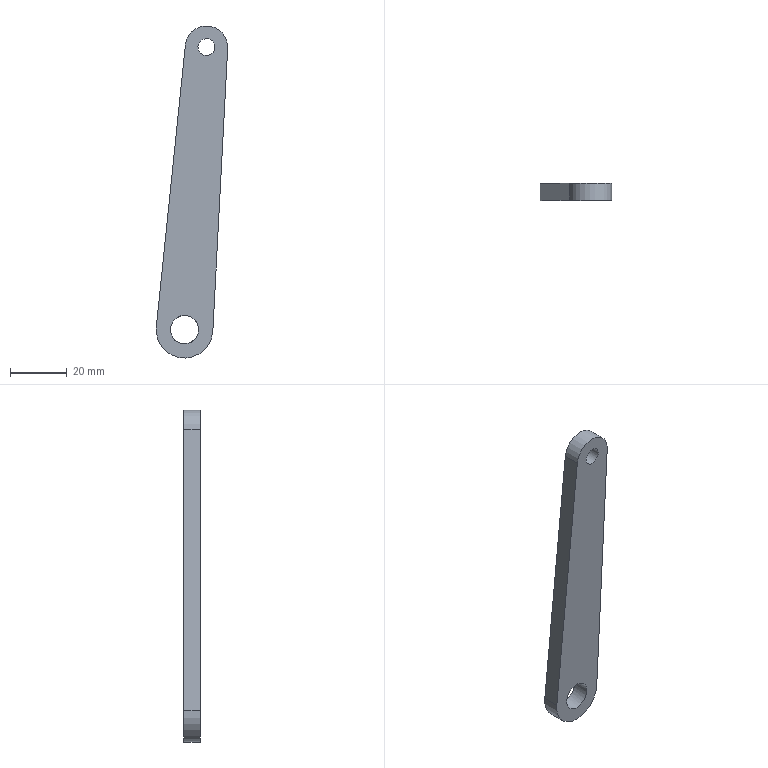Component | NX | CONNECTING_ROD | 1 solid | 8 faces | box 25.25 x 6 x 117.2 mm | volume 11335 mm3 | plane 4 | cylinder 4 | commonest cylinder face diameters 20 x1 15 x1 10 x1 6 x1
STEP:
#1=CARTESIAN_POINT('',(0.,0.,0.));
#2=DIRECTION('',(0.,0.,1.));
#3=DIRECTION('',(1.,0.,0.));
#4=AXIS2_PLACEMENT_3D('',#1,#2,#3);
#5=CARTESIAN_POINT('',(-7.355,48.,110.703));
#6=VERTEX_POINT('',#5);
#7=CARTESIAN_POINT('',(-17.588,48.,11.259));
#8=VERTEX_POINT('',#7);
#9=CARTESIAN_POINT('',(-7.355,48.,110.703));
#10=DIRECTION('',(-0.1024,0.,-0.9947));
#11=VECTOR('',#10,1.);
#12=LINE('',#9,#11);
#13=CARTESIAN_POINT('',(-7.355,42.,110.703));
#14=DIRECTION('',(0.9947,0.,-0.1024));
#15=DIRECTION('',(-0.1024,0.,-0.9947));
#16=AXIS2_PLACEMENT_3D('',#13,#14,#15);
#17=PLANE('',#16);
#18=CARTESIAN_POINT('',(0.,6.));
#19=DIRECTION('',(1.,0.));
#20=VECTOR('',#19,1.);
#21=LINE('',#18,#20);
#22=(GEOMETRIC_REPRESENTATION_CONTEXT(2)PARAMETRIC_REPRESENTATION_CONTEXT()REPRESENTATION_CONTEXT('',''));
#23=DEFINITIONAL_REPRESENTATION('',(#21),#22);
#24=PCURVE('',#17,#23);
#25=CARTESIAN_POINT('',(-7.64,48.,10.235));
#26=DIRECTION('',(0.,-1.,0.));
#27=DIRECTION('',(-0.07746,0.,-0.997));
#28=AXIS2_PLACEMENT_3D('',#25,#26,#27);
#29=PLANE('',#28);
#30=CARTESIAN_POINT('',(-100.188,-7.498));
#31=DIRECTION('',(0.9997,-0.025));
#32=VECTOR('',#31,1.);
#33=LINE('',#30,#32);
#34=(GEOMETRIC_REPRESENTATION_CONTEXT(2)PARAMETRIC_REPRESENTATION_CONTEXT()REPRESENTATION_CONTEXT('',''));
#35=DEFINITIONAL_REPRESENTATION('',(#33),#34);
#36=PCURVE('',#29,#35);
#37=SURFACE_CURVE('',#12,(#24,#36),.PCURVE_S1.);
#38=EDGE_CURVE('',#6,#8,#37,.T.);
#39=ORIENTED_EDGE('',*,*,#38,.T.);
#40=CARTESIAN_POINT('',(-17.588,42.,11.259));
#41=VERTEX_POINT('',#40);
#42=CARTESIAN_POINT('',(-17.588,42.,11.259));
#43=DIRECTION('',(0.,1.,0.));
#44=VECTOR('',#43,1.);
#45=LINE('',#42,#44);
#46=CARTESIAN_POINT('',(99.969,0.));
#47=DIRECTION('',(0.,1.));
#48=VECTOR('',#47,1.);
#49=LINE('',#46,#48);
#50=(GEOMETRIC_REPRESENTATION_CONTEXT(2)PARAMETRIC_REPRESENTATION_CONTEXT()REPRESENTATION_CONTEXT('',''));
#51=DEFINITIONAL_REPRESENTATION('',(#49),#50);
#52=PCURVE('',#17,#51);
#53=CARTESIAN_POINT('',(-7.64,42.,10.235));
#54=DIRECTION('',(0.,1.,0.));
#55=DIRECTION('',(0.07746,0.,0.997));
#56=AXIS2_PLACEMENT_3D('',#53,#54,#55);
#57=CYLINDRICAL_SURFACE('',#56,10.);
#58=CARTESIAN_POINT('',(4.737,0.));
#59=DIRECTION('',(0.,1.));
#60=VECTOR('',#59,1.);
#61=LINE('',#58,#60);
#62=(GEOMETRIC_REPRESENTATION_CONTEXT(2)PARAMETRIC_REPRESENTATION_CONTEXT()REPRESENTATION_CONTEXT('',''));
#63=DEFINITIONAL_REPRESENTATION('',(#61),#62);
#64=PCURVE('',#57,#63);
#65=SURFACE_CURVE('',#45,(#52,#64),.PCURVE_S1.);
#66=EDGE_CURVE('',#41,#8,#65,.T.);
#67=ORIENTED_EDGE('',*,*,#66,.F.);
#68=CARTESIAN_POINT('',(-7.355,42.,110.703));
#69=VERTEX_POINT('',#68);
#70=CARTESIAN_POINT('',(-7.355,42.,110.703));
#71=DIRECTION('',(-0.1024,0.,-0.9947));
#72=VECTOR('',#71,1.);
#73=LINE('',#70,#72);
#74=CARTESIAN_POINT('',(0.,0.));
#75=DIRECTION('',(1.,0.));
#76=VECTOR('',#75,1.);
#77=LINE('',#74,#76);
#78=(GEOMETRIC_REPRESENTATION_CONTEXT(2)PARAMETRIC_REPRESENTATION_CONTEXT()REPRESENTATION_CONTEXT('',''));
#79=DEFINITIONAL_REPRESENTATION('',(#77),#78);
#80=PCURVE('',#17,#79);
#81=CARTESIAN_POINT('',(-7.64,42.,10.235));
#82=DIRECTION('',(0.,-1.,0.));
#83=DIRECTION('',(-0.07746,0.,-0.997));
#84=AXIS2_PLACEMENT_3D('',#81,#82,#83);
#85=PLANE('',#84);
#86=CARTESIAN_POINT('',(-100.188,-7.498));
#87=DIRECTION('',(0.9997,-0.025));
#88=VECTOR('',#87,1.);
#89=LINE('',#86,#88);
#90=(GEOMETRIC_REPRESENTATION_CONTEXT(2)PARAMETRIC_REPRESENTATION_CONTEXT()REPRESENTATION_CONTEXT('',''));
#91=DEFINITIONAL_REPRESENTATION('',(#89),#90);
#92=PCURVE('',#85,#91);
#93=SURFACE_CURVE('',#73,(#80,#92),.PCURVE_S1.);
#94=EDGE_CURVE('',#69,#41,#93,.T.);
#95=ORIENTED_EDGE('',*,*,#94,.F.);
#96=CARTESIAN_POINT('',(-7.355,42.,110.703));
#97=DIRECTION('',(0.,1.,0.));
#98=VECTOR('',#97,1.);
#99=LINE('',#96,#98);
#100=CARTESIAN_POINT('',(0.,0.));
#101=DIRECTION('',(0.,1.));
#102=VECTOR('',#101,1.);
#103=LINE('',#100,#102);
#104=(GEOMETRIC_REPRESENTATION_CONTEXT(2)PARAMETRIC_REPRESENTATION_CONTEXT()REPRESENTATION_CONTEXT('',''));
#105=DEFINITIONAL_REPRESENTATION('',(#103),#104);
#106=PCURVE('',#17,#105);
#107=CARTESIAN_POINT('',(0.1056,42.,109.935));
#108=DIRECTION('',(0.,1.,0.));
#109=DIRECTION('',(0.07746,0.,0.997));
#110=AXIS2_PLACEMENT_3D('',#107,#108,#109);
#111=CYLINDRICAL_SURFACE('',#110,7.5);
#112=CARTESIAN_POINT('',(-1.546,0.));
#113=DIRECTION('',(0.,1.));
#114=VECTOR('',#113,1.);
#115=LINE('',#112,#114);
#116=(GEOMETRIC_REPRESENTATION_CONTEXT(2)PARAMETRIC_REPRESENTATION_CONTEXT()REPRESENTATION_CONTEXT('',''));
#117=DEFINITIONAL_REPRESENTATION('',(#115),#116);
#118=PCURVE('',#111,#117);
#119=SURFACE_CURVE('',#99,(#106,#118),.PCURVE_S1.);
#120=EDGE_CURVE('',#69,#6,#119,.T.);
#121=ORIENTED_EDGE('',*,*,#120,.T.);
#122=EDGE_LOOP('',(#39,#67,#95,#121));
#123=FACE_BOUND('',#122,.T.);
#124=ADVANCED_FACE('',(#123),#17,.F.);
#125=CARTESIAN_POINT('',(2.346,48.,9.71));
#126=VERTEX_POINT('',#125);
#127=CARTESIAN_POINT('',(-7.64,48.,10.235));
#128=DIRECTION('',(0.,-1.,0.));
#129=DIRECTION('',(0.997,0.,-0.07746));
#130=AXIS2_PLACEMENT_3D('',#127,#128,#129);
#131=CIRCLE('',#130,10.);
#132=CARTESIAN_POINT('',(7.854,6.));
#133=DIRECTION('',(-1.,0.));
#134=VECTOR('',#133,1.);
#135=LINE('',#132,#134);
#136=(GEOMETRIC_REPRESENTATION_CONTEXT(2)PARAMETRIC_REPRESENTATION_CONTEXT()REPRESENTATION_CONTEXT('',''));
#137=DEFINITIONAL_REPRESENTATION('',(#135),#136);
#138=PCURVE('',#57,#137);
#139=CARTESIAN_POINT('',(0.,0.));
#140=DIRECTION('',(0.,1.));
#141=AXIS2_PLACEMENT_2D('',#139,#140);
#142=CIRCLE('',#141,10.);
#143=(GEOMETRIC_REPRESENTATION_CONTEXT(2)PARAMETRIC_REPRESENTATION_CONTEXT()REPRESENTATION_CONTEXT('',''));
#144=DEFINITIONAL_REPRESENTATION('',(#142),#143);
#145=PCURVE('',#29,#144);
#146=SURFACE_CURVE('',#131,(#138,#145),.PCURVE_S1.);
#147=EDGE_CURVE('',#8,#126,#146,.T.);
#148=ORIENTED_EDGE('',*,*,#147,.T.);
#149=CARTESIAN_POINT('',(2.346,42.,9.71));
#150=VERTEX_POINT('',#149);
#151=CARTESIAN_POINT('',(2.346,42.,9.71));
#152=DIRECTION('',(0.,1.,0.));
#153=VECTOR('',#152,1.);
#154=LINE('',#151,#153);
#155=CARTESIAN_POINT('',(1.546,0.));
#156=DIRECTION('',(0.,1.));
#157=VECTOR('',#156,1.);
#158=LINE('',#155,#157);
#159=(GEOMETRIC_REPRESENTATION_CONTEXT(2)PARAMETRIC_REPRESENTATION_CONTEXT()REPRESENTATION_CONTEXT('',''));
#160=DEFINITIONAL_REPRESENTATION('',(#158),#159);
#161=PCURVE('',#57,#160);
#162=CARTESIAN_POINT('',(2.346,42.,9.71));
#163=DIRECTION('',(-0.9986,0.,0.05251));
#164=DIRECTION('',(0.05251,0.,0.9986));
#165=AXIS2_PLACEMENT_3D('',#162,#163,#164);
#166=PLANE('',#165);
#167=CARTESIAN_POINT('',(0.,0.));
#168=DIRECTION('',(0.,1.));
#169=VECTOR('',#168,1.);
#170=LINE('',#167,#169);
#171=(GEOMETRIC_REPRESENTATION_CONTEXT(2)PARAMETRIC_REPRESENTATION_CONTEXT()REPRESENTATION_CONTEXT('',''));
#172=DEFINITIONAL_REPRESENTATION('',(#170),#171);
#173=PCURVE('',#166,#172);
#174=SURFACE_CURVE('',#154,(#161,#173),.PCURVE_S1.);
#175=EDGE_CURVE('',#150,#126,#174,.T.);
#176=ORIENTED_EDGE('',*,*,#175,.F.);
#177=CARTESIAN_POINT('',(-7.64,42.,10.235));
#178=DIRECTION('',(0.,-1.,0.));
#179=DIRECTION('',(0.997,0.,-0.07746));
#180=AXIS2_PLACEMENT_3D('',#177,#178,#179);
#181=CIRCLE('',#180,10.);
#182=CARTESIAN_POINT('',(7.854,0.));
#183=DIRECTION('',(-1.,0.));
#184=VECTOR('',#183,1.);
#185=LINE('',#182,#184);
#186=(GEOMETRIC_REPRESENTATION_CONTEXT(2)PARAMETRIC_REPRESENTATION_CONTEXT()REPRESENTATION_CONTEXT('',''));
#187=DEFINITIONAL_REPRESENTATION('',(#185),#186);
#188=PCURVE('',#57,#187);
#189=CARTESIAN_POINT('',(0.,0.));
#190=DIRECTION('',(0.,1.));
#191=AXIS2_PLACEMENT_2D('',#189,#190);
#192=CIRCLE('',#191,10.);
#193=(GEOMETRIC_REPRESENTATION_CONTEXT(2)PARAMETRIC_REPRESENTATION_CONTEXT()REPRESENTATION_CONTEXT('',''));
#194=DEFINITIONAL_REPRESENTATION('',(#192),#193);
#195=PCURVE('',#85,#194);
#196=SURFACE_CURVE('',#181,(#188,#195),.PCURVE_S1.);
#197=EDGE_CURVE('',#41,#150,#196,.T.);
#198=ORIENTED_EDGE('',*,*,#197,.F.);
#199=ORIENTED_EDGE('',*,*,#66,.T.);
#200=EDGE_LOOP('',(#148,#176,#198,#199));
#201=FACE_BOUND('',#200,.T.);
#202=ADVANCED_FACE('',(#201),#57,.T.);
#203=CARTESIAN_POINT('',(7.595,48.,109.541));
#204=VERTEX_POINT('',#203);
#205=CARTESIAN_POINT('',(2.346,48.,9.71));
#206=DIRECTION('',(0.05251,0.,0.9986));
#207=VECTOR('',#206,1.);
#208=LINE('',#205,#207);
#209=CARTESIAN_POINT('',(0.,6.));
#210=DIRECTION('',(1.,0.));
#211=VECTOR('',#210,1.);
#212=LINE('',#209,#211);
#213=(GEOMETRIC_REPRESENTATION_CONTEXT(2)PARAMETRIC_REPRESENTATION_CONTEXT()REPRESENTATION_CONTEXT('',''));
#214=DEFINITIONAL_REPRESENTATION('',(#212),#213);
#215=PCURVE('',#166,#214);
#216=CARTESIAN_POINT('',(-0.25,9.997));
#217=DIRECTION('',(-0.9997,-0.025));
#218=VECTOR('',#217,1.);
#219=LINE('',#216,#218);
#220=(GEOMETRIC_REPRESENTATION_CONTEXT(2)PARAMETRIC_REPRESENTATION_CONTEXT()REPRESENTATION_CONTEXT('',''));
#221=DEFINITIONAL_REPRESENTATION('',(#219),#220);
#222=PCURVE('',#29,#221);
#223=SURFACE_CURVE('',#208,(#215,#222),.PCURVE_S1.);
#224=EDGE_CURVE('',#126,#204,#223,.T.);
#225=ORIENTED_EDGE('',*,*,#224,.T.);
#226=CARTESIAN_POINT('',(7.595,42.,109.541));
#227=VERTEX_POINT('',#226);
#228=CARTESIAN_POINT('',(7.595,42.,109.541));
#229=DIRECTION('',(0.,1.,0.));
#230=VECTOR('',#229,1.);
#231=LINE('',#228,#230);
#232=CARTESIAN_POINT('',(99.969,0.));
#233=DIRECTION('',(0.,1.));
#234=VECTOR('',#233,1.);
#235=LINE('',#232,#234);
#236=(GEOMETRIC_REPRESENTATION_CONTEXT(2)PARAMETRIC_REPRESENTATION_CONTEXT()REPRESENTATION_CONTEXT('',''));
#237=DEFINITIONAL_REPRESENTATION('',(#235),#236);
#238=PCURVE('',#166,#237);
#239=CARTESIAN_POINT('',(1.546,0.));
#240=DIRECTION('',(0.,1.));
#241=VECTOR('',#240,1.);
#242=LINE('',#239,#241);
#243=(GEOMETRIC_REPRESENTATION_CONTEXT(2)PARAMETRIC_REPRESENTATION_CONTEXT()REPRESENTATION_CONTEXT('',''));
#244=DEFINITIONAL_REPRESENTATION('',(#242),#243);
#245=PCURVE('',#111,#244);
#246=SURFACE_CURVE('',#231,(#238,#245),.PCURVE_S1.);
#247=EDGE_CURVE('',#227,#204,#246,.T.);
#248=ORIENTED_EDGE('',*,*,#247,.F.);
#249=CARTESIAN_POINT('',(2.346,42.,9.71));
#250=DIRECTION('',(0.05251,0.,0.9986));
#251=VECTOR('',#250,1.);
#252=LINE('',#249,#251);
#253=CARTESIAN_POINT('',(0.,0.));
#254=DIRECTION('',(1.,0.));
#255=VECTOR('',#254,1.);
#256=LINE('',#253,#255);
#257=(GEOMETRIC_REPRESENTATION_CONTEXT(2)PARAMETRIC_REPRESENTATION_CONTEXT()REPRESENTATION_CONTEXT('',''));
#258=DEFINITIONAL_REPRESENTATION('',(#256),#257);
#259=PCURVE('',#166,#258);
#260=CARTESIAN_POINT('',(-0.25,9.997));
#261=DIRECTION('',(-0.9997,-0.025));
#262=VECTOR('',#261,1.);
#263=LINE('',#260,#262);
#264=(GEOMETRIC_REPRESENTATION_CONTEXT(2)PARAMETRIC_REPRESENTATION_CONTEXT()REPRESENTATION_CONTEXT('',''));
#265=DEFINITIONAL_REPRESENTATION('',(#263),#264);
#266=PCURVE('',#85,#265);
#267=SURFACE_CURVE('',#252,(#259,#266),.PCURVE_S1.);
#268=EDGE_CURVE('',#150,#227,#267,.T.);
#269=ORIENTED_EDGE('',*,*,#268,.F.);
#270=ORIENTED_EDGE('',*,*,#175,.T.);
#271=EDGE_LOOP('',(#225,#248,#269,#270));
#272=FACE_BOUND('',#271,.T.);
#273=ADVANCED_FACE('',(#272),#166,.F.);
#274=CARTESIAN_POINT('',(0.1056,48.,109.935));
#275=DIRECTION('',(0.,-1.,0.));
#276=DIRECTION('',(0.997,0.,-0.07746));
#277=AXIS2_PLACEMENT_3D('',#274,#275,#276);
#278=CIRCLE('',#277,7.5);
#279=CARTESIAN_POINT('',(1.571,6.));
#280=DIRECTION('',(-1.,0.));
#281=VECTOR('',#280,1.);
#282=LINE('',#279,#281);
#283=(GEOMETRIC_REPRESENTATION_CONTEXT(2)PARAMETRIC_REPRESENTATION_CONTEXT()REPRESENTATION_CONTEXT('',''));
#284=DEFINITIONAL_REPRESENTATION('',(#282),#283);
#285=PCURVE('',#111,#284);
#286=CARTESIAN_POINT('',(-100.,0.));
#287=DIRECTION('',(-0.,1.));
#288=AXIS2_PLACEMENT_2D('',#286,#287);
#289=CIRCLE('',#288,7.5);
#290=(GEOMETRIC_REPRESENTATION_CONTEXT(2)PARAMETRIC_REPRESENTATION_CONTEXT()REPRESENTATION_CONTEXT('',''));
#291=DEFINITIONAL_REPRESENTATION('',(#289),#290);
#292=PCURVE('',#29,#291);
#293=SURFACE_CURVE('',#278,(#285,#292),.PCURVE_S1.);
#294=EDGE_CURVE('',#204,#6,#293,.T.);
#295=ORIENTED_EDGE('',*,*,#294,.T.);
#296=ORIENTED_EDGE('',*,*,#120,.F.);
#297=CARTESIAN_POINT('',(0.1056,42.,109.935));
#298=DIRECTION('',(0.,-1.,0.));
#299=DIRECTION('',(0.997,0.,-0.07746));
#300=AXIS2_PLACEMENT_3D('',#297,#298,#299);
#301=CIRCLE('',#300,7.5);
#302=CARTESIAN_POINT('',(1.571,0.));
#303=DIRECTION('',(-1.,0.));
#304=VECTOR('',#303,1.);
#305=LINE('',#302,#304);
#306=(GEOMETRIC_REPRESENTATION_CONTEXT(2)PARAMETRIC_REPRESENTATION_CONTEXT()REPRESENTATION_CONTEXT('',''));
#307=DEFINITIONAL_REPRESENTATION('',(#305),#306);
#308=PCURVE('',#111,#307);
#309=CARTESIAN_POINT('',(-100.,0.));
#310=DIRECTION('',(-0.,1.));
#311=AXIS2_PLACEMENT_2D('',#309,#310);
#312=CIRCLE('',#311,7.5);
#313=(GEOMETRIC_REPRESENTATION_CONTEXT(2)PARAMETRIC_REPRESENTATION_CONTEXT()REPRESENTATION_CONTEXT('',''));
#314=DEFINITIONAL_REPRESENTATION('',(#312),#313);
#315=PCURVE('',#85,#314);
#316=SURFACE_CURVE('',#301,(#308,#315),.PCURVE_S1.);
#317=EDGE_CURVE('',#227,#69,#316,.T.);
#318=ORIENTED_EDGE('',*,*,#317,.F.);
#319=ORIENTED_EDGE('',*,*,#247,.T.);
#320=EDGE_LOOP('',(#295,#296,#318,#319));
#321=FACE_BOUND('',#320,.T.);
#322=ADVANCED_FACE('',(#321),#111,.T.);
#323=CARTESIAN_POINT('',(-0.1268,42.,106.944));
#324=VERTEX_POINT('',#323);
#325=CARTESIAN_POINT('',(-2.885,42.,110.167));
#326=VERTEX_POINT('',#325);
#327=CARTESIAN_POINT('',(0.1056,42.,109.935));
#328=DIRECTION('',(0.,1.,0.));
#329=DIRECTION('',(-0.07746,0.,-0.997));
#330=AXIS2_PLACEMENT_3D('',#327,#328,#329);
#331=CIRCLE('',#330,3.);
#332=CARTESIAN_POINT('',(-97.,0.));
#333=CARTESIAN_POINT('',(-97.,-5.196));
#334=CARTESIAN_POINT('',(-101.5,-2.598));
#335=CARTESIAN_POINT('',(-106.,0.));
#336=CARTESIAN_POINT('',(-101.5,2.598));
#337=CARTESIAN_POINT('',(-97.,5.196));
#338=CARTESIAN_POINT('',(-97.,0.));
#339=(BOUNDED_CURVE()B_SPLINE_CURVE(2,(#332,#333,#334,#335,#336,#337,#338),.UNSPECIFIED.,.T.,.F.)B_SPLINE_CURVE_WITH_KNOTS((1,2,2,2,2,1),(-2.094,0.,2.094,4.189,6.283,8.378),.UNSPECIFIED.)CURVE()GEOMETRIC_REPRESENTATION_ITEM()RATIONAL_B_SPLINE_CURVE((1.,0.5,1.,0.5,1.,0.5,1.))REPRESENTATION_ITEM(''));
#340=(GEOMETRIC_REPRESENTATION_CONTEXT(2)PARAMETRIC_REPRESENTATION_CONTEXT()REPRESENTATION_CONTEXT('',''));
#341=DEFINITIONAL_REPRESENTATION('',(#339),#340);
#342=PCURVE('',#85,#341);
#343=CARTESIAN_POINT('',(0.1056,41.4,109.935));
#344=DIRECTION('',(0.,1.,0.));
#345=DIRECTION('',(0.07746,0.,0.997));
#346=AXIS2_PLACEMENT_3D('',#343,#344,#345);
#347=CYLINDRICAL_SURFACE('',#346,3.);
#348=CARTESIAN_POINT('',(9.425,0.6));
#349=DIRECTION('',(1.,0.));
#350=VECTOR('',#349,1.);
#351=LINE('',#348,#350);
#352=(GEOMETRIC_REPRESENTATION_CONTEXT(2)PARAMETRIC_REPRESENTATION_CONTEXT()REPRESENTATION_CONTEXT('',''));
#353=DEFINITIONAL_REPRESENTATION('',(#351),#352);
#354=PCURVE('',#347,#353);
#355=SURFACE_CURVE('',#331,(#342,#354),.PCURVE_S1.);
#356=EDGE_CURVE('',#324,#326,#355,.T.);
#357=ORIENTED_EDGE('',*,*,#356,.T.);
#358=CARTESIAN_POINT('',(0.1056,42.,109.935));
#359=DIRECTION('',(0.,1.,0.));
#360=DIRECTION('',(-0.07746,0.,-0.997));
#361=AXIS2_PLACEMENT_3D('',#358,#359,#360);
#362=CIRCLE('',#361,3.);
#363=CARTESIAN_POINT('',(-97.,0.));
#364=CARTESIAN_POINT('',(-97.,-5.196));
#365=CARTESIAN_POINT('',(-101.5,-2.598));
#366=CARTESIAN_POINT('',(-106.,0.));
#367=CARTESIAN_POINT('',(-101.5,2.598));
#368=CARTESIAN_POINT('',(-97.,5.196));
#369=CARTESIAN_POINT('',(-97.,0.));
#370=(BOUNDED_CURVE()B_SPLINE_CURVE(2,(#363,#364,#365,#366,#367,#368,#369),.UNSPECIFIED.,.T.,.F.)B_SPLINE_CURVE_WITH_KNOTS((1,2,2,2,2,1),(-2.094,0.,2.094,4.189,6.283,8.378),.UNSPECIFIED.)CURVE()GEOMETRIC_REPRESENTATION_ITEM()RATIONAL_B_SPLINE_CURVE((1.,0.5,1.,0.5,1.,0.5,1.))REPRESENTATION_ITEM(''));
#371=(GEOMETRIC_REPRESENTATION_CONTEXT(2)PARAMETRIC_REPRESENTATION_CONTEXT()REPRESENTATION_CONTEXT('',''));
#372=DEFINITIONAL_REPRESENTATION('',(#370),#371);
#373=PCURVE('',#85,#372);
#374=CARTESIAN_POINT('',(3.142,0.6));
#375=DIRECTION('',(1.,0.));
#376=VECTOR('',#375,1.);
#377=LINE('',#374,#376);
#378=(GEOMETRIC_REPRESENTATION_CONTEXT(2)PARAMETRIC_REPRESENTATION_CONTEXT()REPRESENTATION_CONTEXT('',''));
#379=DEFINITIONAL_REPRESENTATION('',(#377),#378);
#380=PCURVE('',#347,#379);
#381=SURFACE_CURVE('',#362,(#373,#380),.PCURVE_S1.);
#382=EDGE_CURVE('',#326,#324,#381,.T.);
#383=ORIENTED_EDGE('',*,*,#382,.T.);
#384=EDGE_LOOP('',(#357,#383));
#385=FACE_BOUND('',#384,.T.);
#386=CARTESIAN_POINT('',(-8.027,42.,5.25));
#387=VERTEX_POINT('',#386);
#388=CARTESIAN_POINT('',(-12.625,42.,10.623));
#389=VERTEX_POINT('',#388);
#390=CARTESIAN_POINT('',(-7.64,42.,10.235));
#391=DIRECTION('',(0.,1.,0.));
#392=DIRECTION('',(-0.07746,0.,-0.997));
#393=AXIS2_PLACEMENT_3D('',#390,#391,#392);
#394=CIRCLE('',#393,5.);
#395=CARTESIAN_POINT('',(5.,0.));
#396=CARTESIAN_POINT('',(5.,-8.66));
#397=CARTESIAN_POINT('',(-2.5,-4.33));
#398=CARTESIAN_POINT('',(-10.,-0.));
#399=CARTESIAN_POINT('',(-2.5,4.33));
#400=CARTESIAN_POINT('',(5.,8.66));
#401=CARTESIAN_POINT('',(5.,0.));
#402=(BOUNDED_CURVE()B_SPLINE_CURVE(2,(#395,#396,#397,#398,#399,#400,#401),.UNSPECIFIED.,.T.,.F.)B_SPLINE_CURVE_WITH_KNOTS((1,2,2,2,2,1),(-2.094,0.,2.094,4.189,6.283,8.378),.UNSPECIFIED.)CURVE()GEOMETRIC_REPRESENTATION_ITEM()RATIONAL_B_SPLINE_CURVE((1.,0.5,1.,0.5,1.,0.5,1.))REPRESENTATION_ITEM(''));
#403=(GEOMETRIC_REPRESENTATION_CONTEXT(2)PARAMETRIC_REPRESENTATION_CONTEXT()REPRESENTATION_CONTEXT('',''));
#404=DEFINITIONAL_REPRESENTATION('',(#402),#403);
#405=PCURVE('',#85,#404);
#406=CARTESIAN_POINT('',(-7.64,41.4,10.235));
#407=DIRECTION('',(0.,1.,0.));
#408=DIRECTION('',(0.07746,0.,0.997));
#409=AXIS2_PLACEMENT_3D('',#406,#407,#408);
#410=CYLINDRICAL_SURFACE('',#409,5.);
#411=CARTESIAN_POINT('',(9.425,0.6));
#412=DIRECTION('',(1.,0.));
#413=VECTOR('',#412,1.);
#414=LINE('',#411,#413);
#415=(GEOMETRIC_REPRESENTATION_CONTEXT(2)PARAMETRIC_REPRESENTATION_CONTEXT()REPRESENTATION_CONTEXT('',''));
#416=DEFINITIONAL_REPRESENTATION('',(#414),#415);
#417=PCURVE('',#410,#416);
#418=SURFACE_CURVE('',#394,(#405,#417),.PCURVE_S1.);
#419=EDGE_CURVE('',#387,#389,#418,.T.);
#420=ORIENTED_EDGE('',*,*,#419,.T.);
#421=CARTESIAN_POINT('',(-7.64,42.,10.235));
#422=DIRECTION('',(0.,1.,0.));
#423=DIRECTION('',(-0.07746,0.,-0.997));
#424=AXIS2_PLACEMENT_3D('',#421,#422,#423);
#425=CIRCLE('',#424,5.);
#426=CARTESIAN_POINT('',(5.,0.));
#427=CARTESIAN_POINT('',(5.,-8.66));
#428=CARTESIAN_POINT('',(-2.5,-4.33));
#429=CARTESIAN_POINT('',(-10.,-0.));
#430=CARTESIAN_POINT('',(-2.5,4.33));
#431=CARTESIAN_POINT('',(5.,8.66));
#432=CARTESIAN_POINT('',(5.,0.));
#433=(BOUNDED_CURVE()B_SPLINE_CURVE(2,(#426,#427,#428,#429,#430,#431,#432),.UNSPECIFIED.,.T.,.F.)B_SPLINE_CURVE_WITH_KNOTS((1,2,2,2,2,1),(-2.094,0.,2.094,4.189,6.283,8.378),.UNSPECIFIED.)CURVE()GEOMETRIC_REPRESENTATION_ITEM()RATIONAL_B_SPLINE_CURVE((1.,0.5,1.,0.5,1.,0.5,1.))REPRESENTATION_ITEM(''));
#434=(GEOMETRIC_REPRESENTATION_CONTEXT(2)PARAMETRIC_REPRESENTATION_CONTEXT()REPRESENTATION_CONTEXT('',''));
#435=DEFINITIONAL_REPRESENTATION('',(#433),#434);
#436=PCURVE('',#85,#435);
#437=CARTESIAN_POINT('',(3.142,0.6));
#438=DIRECTION('',(1.,0.));
#439=VECTOR('',#438,1.);
#440=LINE('',#437,#439);
#441=(GEOMETRIC_REPRESENTATION_CONTEXT(2)PARAMETRIC_REPRESENTATION_CONTEXT()REPRESENTATION_CONTEXT('',''));
#442=DEFINITIONAL_REPRESENTATION('',(#440),#441);
#443=PCURVE('',#410,#442);
#444=SURFACE_CURVE('',#425,(#436,#443),.PCURVE_S1.);
#445=EDGE_CURVE('',#389,#387,#444,.T.);
#446=ORIENTED_EDGE('',*,*,#445,.T.);
#447=EDGE_LOOP('',(#420,#446));
#448=FACE_BOUND('',#447,.T.);
#449=ORIENTED_EDGE('',*,*,#94,.T.);
#450=ORIENTED_EDGE('',*,*,#197,.T.);
#451=ORIENTED_EDGE('',*,*,#268,.T.);
#452=ORIENTED_EDGE('',*,*,#317,.T.);
#453=EDGE_LOOP('',(#449,#450,#451,#452));
#454=FACE_BOUND('',#453,.T.);
#455=ADVANCED_FACE('',(#385,#448,#454),#85,.T.);
#456=CARTESIAN_POINT('',(-2.885,48.,110.167));
#457=VERTEX_POINT('',#456);
#458=CARTESIAN_POINT('',(0.1056,48.,109.935));
#459=DIRECTION('',(0.,-1.,0.));
#460=DIRECTION('',(-0.997,0.,0.07746));
#461=AXIS2_PLACEMENT_3D('',#458,#459,#460);
#462=CIRCLE('',#461,3.);
#463=CARTESIAN_POINT('',(-100.,0.));
#464=DIRECTION('',(0.,-1.));
#465=AXIS2_PLACEMENT_2D('',#463,#464);
#466=CIRCLE('',#465,3.);
#467=(GEOMETRIC_REPRESENTATION_CONTEXT(2)PARAMETRIC_REPRESENTATION_CONTEXT()REPRESENTATION_CONTEXT('',''));
#468=DEFINITIONAL_REPRESENTATION('',(#466),#467);
#469=PCURVE('',#29,#468);
#470=CARTESIAN_POINT('',(10.996,6.6));
#471=DIRECTION('',(-1.,0.));
#472=VECTOR('',#471,1.);
#473=LINE('',#470,#472);
#474=(GEOMETRIC_REPRESENTATION_CONTEXT(2)PARAMETRIC_REPRESENTATION_CONTEXT()REPRESENTATION_CONTEXT('',''));
#475=DEFINITIONAL_REPRESENTATION('',(#473),#474);
#476=PCURVE('',#347,#475);
#477=SURFACE_CURVE('',#462,(#469,#476),.PCURVE_S1.);
#478=EDGE_CURVE('',#457,#457,#477,.T.);
#479=ORIENTED_EDGE('',*,*,#478,.T.);
#480=EDGE_LOOP('',(#479));
#481=FACE_BOUND('',#480,.T.);
#482=CARTESIAN_POINT('',(-12.625,48.,10.623));
#483=VERTEX_POINT('',#482);
#484=CARTESIAN_POINT('',(-7.64,48.,10.235));
#485=DIRECTION('',(0.,-1.,0.));
#486=DIRECTION('',(-0.997,0.,0.07746));
#487=AXIS2_PLACEMENT_3D('',#484,#485,#486);
#488=CIRCLE('',#487,5.);
#489=CARTESIAN_POINT('',(0.,0.));
#490=DIRECTION('',(0.,-1.));
#491=AXIS2_PLACEMENT_2D('',#489,#490);
#492=CIRCLE('',#491,5.);
#493=(GEOMETRIC_REPRESENTATION_CONTEXT(2)PARAMETRIC_REPRESENTATION_CONTEXT()REPRESENTATION_CONTEXT('',''));
#494=DEFINITIONAL_REPRESENTATION('',(#492),#493);
#495=PCURVE('',#29,#494);
#496=CARTESIAN_POINT('',(10.996,6.6));
#497=DIRECTION('',(-1.,0.));
#498=VECTOR('',#497,1.);
#499=LINE('',#496,#498);
#500=(GEOMETRIC_REPRESENTATION_CONTEXT(2)PARAMETRIC_REPRESENTATION_CONTEXT()REPRESENTATION_CONTEXT('',''));
#501=DEFINITIONAL_REPRESENTATION('',(#499),#500);
#502=PCURVE('',#410,#501);
#503=SURFACE_CURVE('',#488,(#495,#502),.PCURVE_S1.);
#504=EDGE_CURVE('',#483,#483,#503,.T.);
#505=ORIENTED_EDGE('',*,*,#504,.T.);
#506=EDGE_LOOP('',(#505));
#507=FACE_BOUND('',#506,.T.);
#508=ORIENTED_EDGE('',*,*,#38,.F.);
#509=ORIENTED_EDGE('',*,*,#294,.F.);
#510=ORIENTED_EDGE('',*,*,#224,.F.);
#511=ORIENTED_EDGE('',*,*,#147,.F.);
#512=EDGE_LOOP('',(#508,#509,#510,#511));
#513=FACE_BOUND('',#512,.T.);
#514=ADVANCED_FACE('',(#481,#507,#513),#29,.F.);
#515=ORIENTED_EDGE('',*,*,#419,.T.);
#516=CARTESIAN_POINT('',(-12.625,42.,10.623));
#517=CARTESIAN_POINT('',(-12.625,48.,10.623));
#518=B_SPLINE_CURVE_WITH_KNOTS('',1,(#516,#517),.UNSPECIFIED.,.F.,.F.,(2,2),(0.6,6.6),.PIECEWISE_BEZIER_KNOTS.);
#519=CARTESIAN_POINT('',(10.996,0.));
#520=DIRECTION('',(0.,1.));
#521=VECTOR('',#520,1.);
#522=LINE('',#519,#521);
#523=(GEOMETRIC_REPRESENTATION_CONTEXT(2)PARAMETRIC_REPRESENTATION_CONTEXT()REPRESENTATION_CONTEXT('',''));
#524=DEFINITIONAL_REPRESENTATION('',(#522),#523);
#525=PCURVE('',#410,#524);
#526=CARTESIAN_POINT('',(4.712,0.));
#527=DIRECTION('',(0.,1.));
#528=VECTOR('',#527,1.);
#529=LINE('',#526,#528);
#530=(GEOMETRIC_REPRESENTATION_CONTEXT(2)PARAMETRIC_REPRESENTATION_CONTEXT()REPRESENTATION_CONTEXT('',''));
#531=DEFINITIONAL_REPRESENTATION('',(#529),#530);
#532=PCURVE('',#410,#531);
#533=SEAM_CURVE('',#518,(#525,#532),.PCURVE_S1.);
#534=EDGE_CURVE('',#389,#483,#533,.T.);
#535=ORIENTED_EDGE('',*,*,#534,.T.);
#536=ORIENTED_EDGE('',*,*,#504,.T.);
#537=ORIENTED_EDGE('',*,*,#534,.F.);
#538=ORIENTED_EDGE('',*,*,#445,.T.);
#539=EDGE_LOOP('',(#515,#535,#536,#537,#538));
#540=FACE_BOUND('',#539,.F.);
#541=ADVANCED_FACE('',(#540),#410,.F.);
#542=ORIENTED_EDGE('',*,*,#356,.T.);
#543=CARTESIAN_POINT('',(-2.885,42.,110.167));
#544=CARTESIAN_POINT('',(-2.885,48.,110.167));
#545=B_SPLINE_CURVE_WITH_KNOTS('',1,(#543,#544),.UNSPECIFIED.,.F.,.F.,(2,2),(0.6,6.6),.PIECEWISE_BEZIER_KNOTS.);
#546=CARTESIAN_POINT('',(10.996,0.));
#547=DIRECTION('',(0.,1.));
#548=VECTOR('',#547,1.);
#549=LINE('',#546,#548);
#550=(GEOMETRIC_REPRESENTATION_CONTEXT(2)PARAMETRIC_REPRESENTATION_CONTEXT()REPRESENTATION_CONTEXT('',''));
#551=DEFINITIONAL_REPRESENTATION('',(#549),#550);
#552=PCURVE('',#347,#551);
#553=CARTESIAN_POINT('',(4.712,0.));
#554=DIRECTION('',(0.,1.));
#555=VECTOR('',#554,1.);
#556=LINE('',#553,#555);
#557=(GEOMETRIC_REPRESENTATION_CONTEXT(2)PARAMETRIC_REPRESENTATION_CONTEXT()REPRESENTATION_CONTEXT('',''));
#558=DEFINITIONAL_REPRESENTATION('',(#556),#557);
#559=PCURVE('',#347,#558);
#560=SEAM_CURVE('',#545,(#552,#559),.PCURVE_S1.);
#561=EDGE_CURVE('',#326,#457,#560,.T.);
#562=ORIENTED_EDGE('',*,*,#561,.T.);
#563=ORIENTED_EDGE('',*,*,#478,.T.);
#564=ORIENTED_EDGE('',*,*,#561,.F.);
#565=ORIENTED_EDGE('',*,*,#382,.T.);
#566=EDGE_LOOP('',(#542,#562,#563,#564,#565));
#567=FACE_BOUND('',#566,.F.);
#568=ADVANCED_FACE('',(#567),#347,.F.);
#569=CLOSED_SHELL('',(#124,#202,#273,#322,#455,#514,#541,#568));
#570=MANIFOLD_SOLID_BREP('',#569);
#571=(LENGTH_UNIT()NAMED_UNIT(*)SI_UNIT(.MILLI.,.METRE.));
#572=UNCERTAINTY_MEASURE_WITH_UNIT(LENGTH_MEASURE(0.000002),#571,'','');
#573=(NAMED_UNIT(*)PLANE_ANGLE_UNIT()SI_UNIT($,.RADIAN.));
#574=(NAMED_UNIT(*)SI_UNIT($,.STERADIAN.)SOLID_ANGLE_UNIT());
#575=(GEOMETRIC_REPRESENTATION_CONTEXT(3)GLOBAL_UNCERTAINTY_ASSIGNED_CONTEXT((#572))GLOBAL_UNIT_ASSIGNED_CONTEXT((#571,#573,#574))REPRESENTATION_CONTEXT('',''));
#576=ADVANCED_BREP_SHAPE_REPRESENTATION('',(#4,#570),#575);